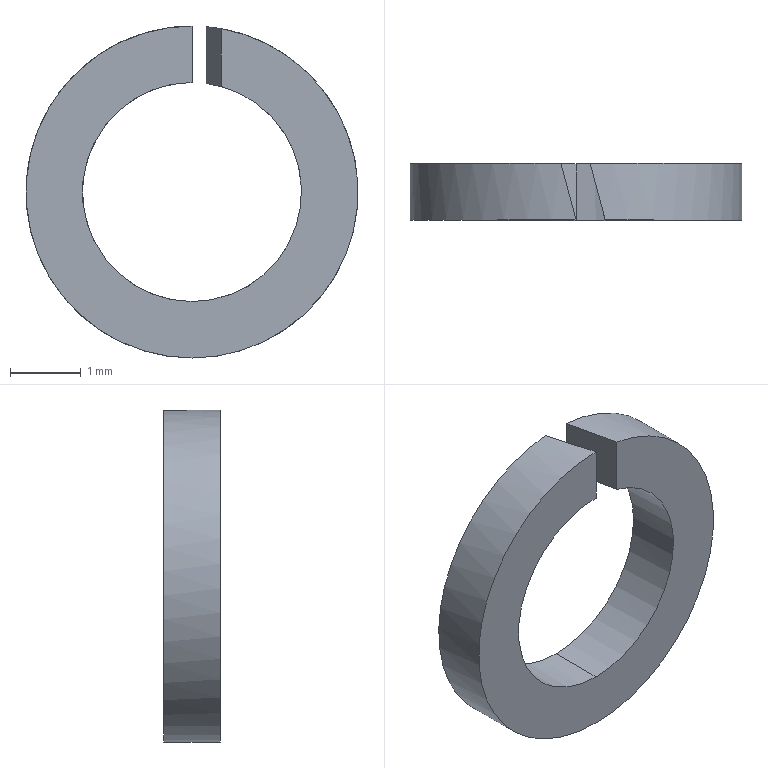Component | SolidWorks | GB 93-87-3-11 | 1 solid | 8 faces | box 4.7 x 0.8 x 4.7 mm | volume 8 mm3 | cylinder 4 | plane 4 | commonest cylinder face diameters 3.1 x2 4.7 x2
build123d program:
from build123d import *

# Parameters (mm, degrees)
SKETCH1_R               = 2.35
SKETCH1_R_2             = 1.55
BOSS_EXTRUDE1_DEPTH     = 0.8
CUT_EXTRUDE1_REACH      = 5.418
CUT_EXTRUDE1_END_RADIUS = 2.35


with BuildPart() as part:
    # Sketch1 → Boss-Extrude1 (new body)
    with BuildSketch(Plane(origin=(0, 0, 0), x_dir=(1, 0, 0), z_dir=(0, 1, 0))):
        with Locations(Location((0, 0, 0), (0, 0, 270))):
            Circle(SKETCH1_R)
        with Locations(Location((0, 0, 0), (0, 0, 270))):
            Circle(SKETCH1_R_2, mode=Mode.SUBTRACT)
    extrude(amount=BOSS_EXTRUDE1_DEPTH)

    # Cut-Extrude1: up to this cylinder (the profile starts inside it)
    cut_extrude1_end = Plane(origin=(0, 0.4, 0), z_dir=(0, -1, 0)) * Cylinder(CUT_EXTRUDE1_END_RADIUS, 16.536, mode=Mode.PRIVATE)
    # Sketch2 → Cut-Extrude1 (cut, up to the surface)
    with BuildSketch(Plane.XY, mode=Mode.PRIVATE) as cut_extrude1_sk1:
        Polygon((0, 0), (-0.2144, 0.8), (0.1998, 0.8), (0.4141, 0), align=None)
    cut_extrude1_tool1 = extrude(cut_extrude1_sk1.sketch, amount=CUT_EXTRUDE1_REACH, mode=Mode.PRIVATE) & cut_extrude1_end
    add(cut_extrude1_tool1.solids().sort_by_distance((0.09988, 0.4, 0))[0], mode=Mode.SUBTRACT)


solid = part.part

# Placed as in the assembly
solid = solid.moved(Location((-199.914, 44.966, -166.507), (0, 0, 0)))